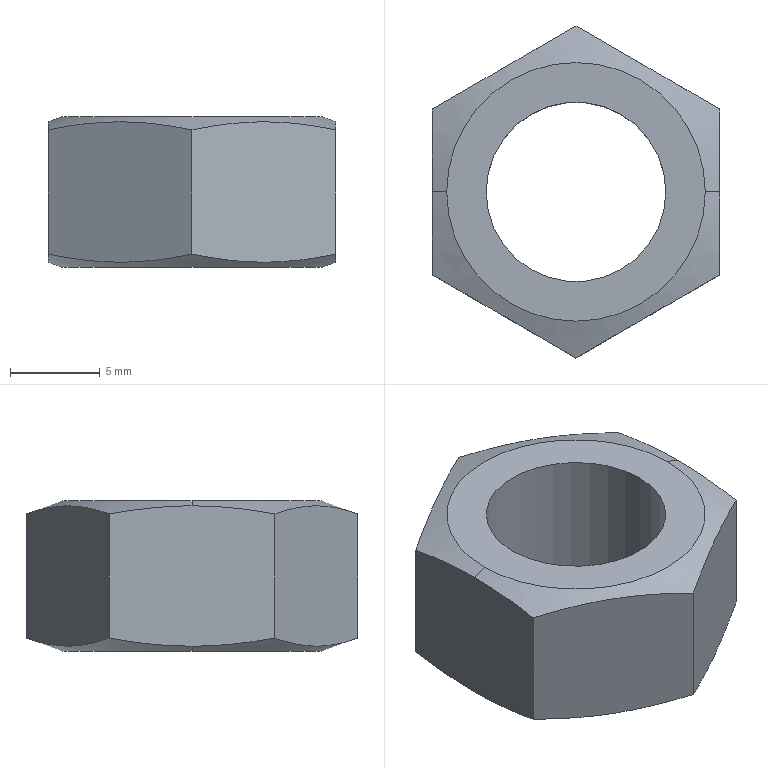Component | SolidWorks | HexNutM10-11 | 1 solid | 14 faces | box 16 x 18.48 x 8.4 mm | volume 1174 mm3 | plane 8 | cone 4 | cylinder 2 | commonest cylinder face diameters 10 x2
build123d program:
from build123d import *

# Parameters (mm, degrees)
BOSS_EXTRUDE1_DEPTH = 8.4
SKETCH5_R           = 5
CUT_EXTRUDE1_DEPTH  = 15.829


with BuildPart() as part:
    # Sketch1 → Boss-Extrude1 (new body)
    with BuildSketch(Plane.XY):
        Polygon((0, 9.238), (-8, 4.619), (-8, -4.619), (0, -9.238), (8, -4.619), (8, 4.619), align=None)
    extrude(amount=BOSS_EXTRUDE1_DEPTH)

    # Sketch4 → Cut-Revolve1 (revolve, cut)
    with BuildSketch(Plane(origin=(0, 0, 0), x_dir=(0, 0, -1), z_dir=(1, 0, 0)), mode=Mode.PRIVATE) as cut_revolve1_sk:
        Polygon((-8.4, -7.2), (-7.658, -9.238), (-8.4, -9.238), align=None)
    cut_revolve1 = revolve(cut_revolve1_sk.sketch.rotate(Axis((0, 0, 8.4), (0, 0, -1)), 120), axis=Axis((0, 0, 8.4), (0, 0, -1)), mode=Mode.SUBTRACT)

    # Mirror1: Cut-Revolve1 across plane
    add(cut_revolve1.mirror(Plane.XY.offset(4.2)), mode=Mode.SUBTRACT)

    # Sketch5 → Cut-Extrude1 (cut, through all)
    with BuildSketch(Plane.XY.offset(8.4)):
        Circle(SKETCH5_R)
    extrude(amount=-CUT_EXTRUDE1_DEPTH, mode=Mode.SUBTRACT)


solid = part.part

# Placed as in the assembly
solid = solid.moved(Location((-5489.995, 7146.665, 122.592), (0, 0, 0)))
STEP:
#1=COLOUR_RGB('',0.7922,0.8196,0.9333);
#2=FILL_AREA_STYLE_COLOUR('',#1);
#3=FILL_AREA_STYLE('',(#2));
#4=SURFACE_STYLE_FILL_AREA(#3);
#5=SURFACE_SIDE_STYLE('',(#4));
#6=SURFACE_STYLE_USAGE(.BOTH.,#5);
#7=PRESENTATION_STYLE_ASSIGNMENT((#6));
#8=CARTESIAN_POINT('',(-216.338,281.365,4.826));
#9=VERTEX_POINT('',#8);
#10=CARTESIAN_POINT('',(-215.945,281.365,4.826));
#11=VERTEX_POINT('',#10);
#12=CARTESIAN_POINT('',(-216.142,281.365,4.826));
#13=DIRECTION('',(0.,0.,1.));
#14=DIRECTION('',(1.,0.,0.));
#15=AXIS2_PLACEMENT_3D('',#12,#13,#14);
#16=CIRCLE('',#15,0.1969);
#17=EDGE_CURVE('',#9,#11,#16,.T.);
#18=ORIENTED_EDGE('',*,*,#17,.F.);
#19=CARTESIAN_POINT('',(-216.338,281.365,5.157));
#20=VERTEX_POINT('',#19);
#21=CARTESIAN_POINT('',(-216.338,281.365,4.826));
#22=DIRECTION('',(0.,0.,1.));
#23=VECTOR('',#22,39.37);
#24=LINE('',#21,#23);
#25=EDGE_CURVE('',#9,#20,#24,.T.);
#26=ORIENTED_EDGE('',*,*,#25,.T.);
#27=CARTESIAN_POINT('',(-215.945,281.365,5.157));
#28=VERTEX_POINT('',#27);
#29=CARTESIAN_POINT('',(-216.142,281.365,5.157));
#30=DIRECTION('',(0.,0.,1.));
#31=DIRECTION('',(1.,0.,0.));
#32=AXIS2_PLACEMENT_3D('',#29,#30,#31);
#33=CIRCLE('',#32,0.1969);
#34=EDGE_CURVE('',#20,#28,#33,.T.);
#35=ORIENTED_EDGE('',*,*,#34,.T.);
#36=CARTESIAN_POINT('',(-215.945,281.365,4.826));
#37=DIRECTION('',(0.,0.,1.));
#38=VECTOR('',#37,39.37);
#39=LINE('',#36,#38);
#40=EDGE_CURVE('',#11,#28,#39,.T.);
#41=ORIENTED_EDGE('',*,*,#40,.F.);
#42=EDGE_LOOP('',(#18,#26,#35,#41));
#43=FACE_OUTER_BOUND('',#42,.T.);
#44=CARTESIAN_POINT('',(-216.142,281.365,4.826));
#45=DIRECTION('',(0.,0.,1.));
#46=DIRECTION('',(1.,0.,0.));
#47=AXIS2_PLACEMENT_3D('',#44,#45,#46);
#48=CYLINDRICAL_SURFACE('',#47,0.1969);
#49=ADVANCED_FACE('',(#43),#48,.F.);
#50=CARTESIAN_POINT('',(-216.425,281.365,4.826));
#51=VERTEX_POINT('',#50);
#52=CARTESIAN_POINT('',(-215.858,281.365,4.826));
#53=VERTEX_POINT('',#52);
#54=CARTESIAN_POINT('',(-216.142,281.365,4.826));
#55=DIRECTION('',(0.,0.,1.));
#56=DIRECTION('',(1.,0.,0.));
#57=AXIS2_PLACEMENT_3D('',#54,#55,#56);
#58=CIRCLE('',#57,0.2835);
#59=EDGE_CURVE('',#51,#53,#58,.T.);
#60=ORIENTED_EDGE('',*,*,#59,.T.);
#61=CARTESIAN_POINT('',(-215.827,281.365,4.838));
#62=VERTEX_POINT('',#61);
#63=CARTESIAN_POINT('',(-215.778,281.365,4.856));
#64=DIRECTION('',(0.9397,-0.,0.342));
#65=VECTOR('',#64,39.37);
#66=LINE('',#63,#65);
#67=EDGE_CURVE('',#53,#62,#66,.T.);
#68=ORIENTED_EDGE('',*,*,#67,.T.);
#69=CARTESIAN_POINT('',(-215.827,281.183,4.856));
#70=VERTEX_POINT('',#69);
#71=CARTESIAN_POINT('',(-215.827,281.183,4.856));
#72=CARTESIAN_POINT('',(-215.827,281.213,4.85));
#73=CARTESIAN_POINT('',(-215.827,281.243,4.846));
#74=CARTESIAN_POINT('',(-215.827,281.304,4.84));
#75=CARTESIAN_POINT('',(-215.827,281.334,4.838));
#76=CARTESIAN_POINT('',(-215.827,281.365,4.838));
#77=B_SPLINE_CURVE_WITH_KNOTS('',3,(#71,#72,#73,#74,#75,#76),.UNSPECIFIED.,.F.,.F.,(4,2,4),(0.007828,0.01016,0.01248),.UNSPECIFIED.);
#78=EDGE_CURVE('',#70,#62,#77,.T.);
#79=ORIENTED_EDGE('',*,*,#78,.F.);
#80=CARTESIAN_POINT('',(-216.142,281.001,4.856));
#81=VERTEX_POINT('',#80);
#82=CARTESIAN_POINT('',(-216.142,281.001,4.856));
#83=CARTESIAN_POINT('',(-216.115,281.016,4.85));
#84=CARTESIAN_POINT('',(-216.089,281.031,4.846));
#85=CARTESIAN_POINT('',(-216.037,281.062,4.84));
#86=CARTESIAN_POINT('',(-215.984,281.092,4.836));
#87=CARTESIAN_POINT('',(-215.932,281.122,4.84));
#88=CARTESIAN_POINT('',(-215.879,281.153,4.846));
#89=CARTESIAN_POINT('',(-215.853,281.168,4.85));
#90=CARTESIAN_POINT('',(-215.827,281.183,4.856));
#91=B_SPLINE_CURVE_WITH_KNOTS('',3,(#82,#83,#84,#85,#86,#87,#88,#89,#90),.UNSPECIFIED.,.F.,.F.,(4,2,1,2,4),(0.00000023,0.00231,0.004619,0.006928,0.009238),.UNSPECIFIED.);
#92=EDGE_CURVE('',#81,#70,#91,.T.);
#93=ORIENTED_EDGE('',*,*,#92,.F.);
#94=CARTESIAN_POINT('',(-216.456,281.183,4.856));
#95=VERTEX_POINT('',#94);
#96=CARTESIAN_POINT('',(-216.456,281.183,4.856));
#97=CARTESIAN_POINT('',(-216.43,281.168,4.85));
#98=CARTESIAN_POINT('',(-216.404,281.153,4.846));
#99=CARTESIAN_POINT('',(-216.351,281.122,4.84));
#100=CARTESIAN_POINT('',(-216.299,281.092,4.836));
#101=CARTESIAN_POINT('',(-216.247,281.062,4.84));
#102=CARTESIAN_POINT('',(-216.194,281.031,4.846));
#103=CARTESIAN_POINT('',(-216.168,281.016,4.85));
#104=CARTESIAN_POINT('',(-216.142,281.001,4.856));
#105=B_SPLINE_CURVE_WITH_KNOTS('',3,(#96,#97,#98,#99,#100,#101,#102,#103,#104),.UNSPECIFIED.,.F.,.F.,(4,2,1,2,4),(0.00000023,0.00231,0.004619,0.006928,0.009238),.UNSPECIFIED.);
#106=EDGE_CURVE('',#95,#81,#105,.T.);
#107=ORIENTED_EDGE('',*,*,#106,.F.);
#108=CARTESIAN_POINT('',(-216.456,281.365,4.838));
#109=VERTEX_POINT('',#108);
#110=CARTESIAN_POINT('',(-216.456,281.365,4.838));
#111=CARTESIAN_POINT('',(-216.456,281.334,4.838));
#112=CARTESIAN_POINT('',(-216.456,281.304,4.84));
#113=CARTESIAN_POINT('',(-216.456,281.243,4.846));
#114=CARTESIAN_POINT('',(-216.456,281.213,4.85));
#115=CARTESIAN_POINT('',(-216.456,281.183,4.856));
#116=B_SPLINE_CURVE_WITH_KNOTS('',3,(#110,#111,#112,#113,#114,#115),.UNSPECIFIED.,.F.,.F.,(4,2,4),(0.02142,0.02374,0.02606),.UNSPECIFIED.);
#117=EDGE_CURVE('',#109,#95,#116,.T.);
#118=ORIENTED_EDGE('',*,*,#117,.F.);
#119=CARTESIAN_POINT('',(-216.505,281.365,4.856));
#120=DIRECTION('',(-0.9397,0.,0.342));
#121=VECTOR('',#120,39.37);
#122=LINE('',#119,#121);
#123=EDGE_CURVE('',#51,#109,#122,.T.);
#124=ORIENTED_EDGE('',*,*,#123,.F.);
#125=EDGE_LOOP('',(#60,#68,#79,#93,#107,#118,#124));
#126=FACE_OUTER_BOUND('',#125,.T.);
#127=CARTESIAN_POINT('',(-216.142,281.365,4.856));
#128=DIRECTION('',(0.,0.,1.));
#129=DIRECTION('',(-1.,0.,0.));
#130=AXIS2_PLACEMENT_3D('',#127,#128,#129);
#131=CONICAL_SURFACE('',#130,0.3637,1.222);
#132=ADVANCED_FACE('',(#126),#131,.T.);
#133=CARTESIAN_POINT('',(-215.858,281.365,5.157));
#134=VERTEX_POINT('',#133);
#135=CARTESIAN_POINT('',(-216.425,281.365,5.157));
#136=VERTEX_POINT('',#135);
#137=CARTESIAN_POINT('',(-216.142,281.365,5.157));
#138=DIRECTION('',(0.,0.,1.));
#139=DIRECTION('',(1.,0.,0.));
#140=AXIS2_PLACEMENT_3D('',#137,#138,#139);
#141=CIRCLE('',#140,0.2835);
#142=EDGE_CURVE('',#134,#136,#141,.T.);
#143=ORIENTED_EDGE('',*,*,#142,.F.);
#144=CARTESIAN_POINT('',(-215.827,281.365,5.146));
#145=VERTEX_POINT('',#144);
#146=CARTESIAN_POINT('',(-215.778,281.365,5.128));
#147=DIRECTION('',(0.9397,0.,-0.342));
#148=VECTOR('',#147,39.37);
#149=LINE('',#146,#148);
#150=EDGE_CURVE('',#134,#145,#149,.T.);
#151=ORIENTED_EDGE('',*,*,#150,.T.);
#152=CARTESIAN_POINT('',(-215.827,281.547,5.128));
#153=VERTEX_POINT('',#152);
#154=CARTESIAN_POINT('',(-215.827,281.547,5.128));
#155=CARTESIAN_POINT('',(-215.827,281.516,5.133));
#156=CARTESIAN_POINT('',(-215.827,281.486,5.138));
#157=CARTESIAN_POINT('',(-215.827,281.425,5.144));
#158=CARTESIAN_POINT('',(-215.827,281.395,5.146));
#159=CARTESIAN_POINT('',(-215.827,281.365,5.146));
#160=B_SPLINE_CURVE_WITH_KNOTS('',3,(#154,#155,#156,#157,#158,#159),.UNSPECIFIED.,.F.,.F.,(4,2,4),(0.01676,0.01909,0.02142),.UNSPECIFIED.);
#161=EDGE_CURVE('',#153,#145,#160,.T.);
#162=ORIENTED_EDGE('',*,*,#161,.F.);
#163=CARTESIAN_POINT('',(-216.142,281.728,5.128));
#164=VERTEX_POINT('',#163);
#165=CARTESIAN_POINT('',(-216.142,281.728,5.128));
#166=CARTESIAN_POINT('',(-216.115,281.713,5.133));
#167=CARTESIAN_POINT('',(-216.089,281.698,5.138));
#168=CARTESIAN_POINT('',(-216.037,281.668,5.144));
#169=CARTESIAN_POINT('',(-215.984,281.638,5.147));
#170=CARTESIAN_POINT('',(-215.932,281.607,5.144));
#171=CARTESIAN_POINT('',(-215.879,281.577,5.138));
#172=CARTESIAN_POINT('',(-215.853,281.562,5.133));
#173=CARTESIAN_POINT('',(-215.827,281.547,5.128));
#174=B_SPLINE_CURVE_WITH_KNOTS('',3,(#165,#166,#167,#168,#169,#170,#171,#172,#173),.UNSPECIFIED.,.F.,.F.,(4,2,1,2,4),(0.00000023,0.00231,0.004619,0.006928,0.009238),.UNSPECIFIED.);
#175=EDGE_CURVE('',#164,#153,#174,.T.);
#176=ORIENTED_EDGE('',*,*,#175,.F.);
#177=CARTESIAN_POINT('',(-216.456,281.547,5.128));
#178=VERTEX_POINT('',#177);
#179=CARTESIAN_POINT('',(-216.456,281.547,5.128));
#180=CARTESIAN_POINT('',(-216.43,281.562,5.133));
#181=CARTESIAN_POINT('',(-216.404,281.577,5.138));
#182=CARTESIAN_POINT('',(-216.351,281.607,5.144));
#183=CARTESIAN_POINT('',(-216.299,281.638,5.147));
#184=CARTESIAN_POINT('',(-216.247,281.668,5.144));
#185=CARTESIAN_POINT('',(-216.194,281.698,5.138));
#186=CARTESIAN_POINT('',(-216.168,281.713,5.133));
#187=CARTESIAN_POINT('',(-216.142,281.728,5.128));
#188=B_SPLINE_CURVE_WITH_KNOTS('',3,(#179,#180,#181,#182,#183,#184,#185,#186,#187),.UNSPECIFIED.,.F.,.F.,(4,2,1,2,4),(0.00000023,0.00231,0.004619,0.006928,0.009238),.UNSPECIFIED.);
#189=EDGE_CURVE('',#178,#164,#188,.T.);
#190=ORIENTED_EDGE('',*,*,#189,.F.);
#191=CARTESIAN_POINT('',(-216.456,281.365,5.146));
#192=VERTEX_POINT('',#191);
#193=CARTESIAN_POINT('',(-216.456,281.365,5.146));
#194=CARTESIAN_POINT('',(-216.456,281.395,5.146));
#195=CARTESIAN_POINT('',(-216.456,281.425,5.144));
#196=CARTESIAN_POINT('',(-216.456,281.486,5.138));
#197=CARTESIAN_POINT('',(-216.456,281.516,5.133));
#198=CARTESIAN_POINT('',(-216.456,281.547,5.128));
#199=B_SPLINE_CURVE_WITH_KNOTS('',3,(#193,#194,#195,#196,#197,#198),.UNSPECIFIED.,.F.,.F.,(4,2,4),(0.01248,0.01482,0.01715),.UNSPECIFIED.);
#200=EDGE_CURVE('',#192,#178,#199,.T.);
#201=ORIENTED_EDGE('',*,*,#200,.F.);
#202=CARTESIAN_POINT('',(-216.505,281.365,5.128));
#203=DIRECTION('',(-0.9397,0.,-0.342));
#204=VECTOR('',#203,39.37);
#205=LINE('',#202,#204);
#206=EDGE_CURVE('',#136,#192,#205,.T.);
#207=ORIENTED_EDGE('',*,*,#206,.F.);
#208=EDGE_LOOP('',(#143,#151,#162,#176,#190,#201,#207));
#209=FACE_OUTER_BOUND('',#208,.T.);
#210=CARTESIAN_POINT('',(-216.142,281.365,5.128));
#211=DIRECTION('',(0.,0.,-1.));
#212=DIRECTION('',(-1.,0.,0.));
#213=AXIS2_PLACEMENT_3D('',#210,#211,#212);
#214=CONICAL_SURFACE('',#213,0.3637,1.222);
#215=ADVANCED_FACE('',(#209),#214,.T.);
#216=CARTESIAN_POINT('',(-215.827,281.547,4.856));
#217=VERTEX_POINT('',#216);
#218=CARTESIAN_POINT('',(-215.827,281.547,5.157));
#219=DIRECTION('',(0.,0.,-1.));
#220=VECTOR('',#219,39.37);
#221=LINE('',#218,#220);
#222=EDGE_CURVE('',#153,#217,#221,.T.);
#223=ORIENTED_EDGE('',*,*,#222,.T.);
#224=CARTESIAN_POINT('',(-216.142,281.728,4.856));
#225=VERTEX_POINT('',#224);
#226=CARTESIAN_POINT('',(-215.827,281.547,4.856));
#227=CARTESIAN_POINT('',(-215.853,281.562,4.85));
#228=CARTESIAN_POINT('',(-215.879,281.577,4.846));
#229=CARTESIAN_POINT('',(-215.932,281.607,4.84));
#230=CARTESIAN_POINT('',(-215.984,281.638,4.836));
#231=CARTESIAN_POINT('',(-216.037,281.668,4.84));
#232=CARTESIAN_POINT('',(-216.089,281.698,4.846));
#233=CARTESIAN_POINT('',(-216.115,281.713,4.85));
#234=CARTESIAN_POINT('',(-216.142,281.728,4.856));
#235=B_SPLINE_CURVE_WITH_KNOTS('',3,(#226,#227,#228,#229,#230,#231,#232,#233,#234),.UNSPECIFIED.,.F.,.F.,(4,2,1,2,4),(0.00000023,0.00231,0.004619,0.006928,0.009238),.UNSPECIFIED.);
#236=EDGE_CURVE('',#217,#225,#235,.T.);
#237=ORIENTED_EDGE('',*,*,#236,.T.);
#238=CARTESIAN_POINT('',(-216.142,281.728,5.157));
#239=DIRECTION('',(0.,0.,-1.));
#240=VECTOR('',#239,39.37);
#241=LINE('',#238,#240);
#242=EDGE_CURVE('',#164,#225,#241,.T.);
#243=ORIENTED_EDGE('',*,*,#242,.F.);
#244=ORIENTED_EDGE('',*,*,#175,.T.);
#245=EDGE_LOOP('',(#223,#237,#243,#244));
#246=FACE_OUTER_BOUND('',#245,.T.);
#247=CARTESIAN_POINT('',(-215.827,281.547,5.157));
#248=DIRECTION('',(-0.5,-0.866,0.));
#249=DIRECTION('',(0.866,-0.5,0.));
#250=AXIS2_PLACEMENT_3D('',#247,#248,#249);
#251=PLANE('',#250);
#252=ADVANCED_FACE('',(#246),#251,.F.);
#253=ORIENTED_EDGE('',*,*,#242,.T.);
#254=CARTESIAN_POINT('',(-216.456,281.547,4.856));
#255=VERTEX_POINT('',#254);
#256=CARTESIAN_POINT('',(-216.142,281.728,4.856));
#257=CARTESIAN_POINT('',(-216.168,281.713,4.85));
#258=CARTESIAN_POINT('',(-216.194,281.698,4.846));
#259=CARTESIAN_POINT('',(-216.247,281.668,4.84));
#260=CARTESIAN_POINT('',(-216.299,281.638,4.836));
#261=CARTESIAN_POINT('',(-216.351,281.607,4.84));
#262=CARTESIAN_POINT('',(-216.404,281.577,4.846));
#263=CARTESIAN_POINT('',(-216.43,281.562,4.85));
#264=CARTESIAN_POINT('',(-216.456,281.547,4.856));
#265=B_SPLINE_CURVE_WITH_KNOTS('',3,(#256,#257,#258,#259,#260,#261,#262,#263,#264),.UNSPECIFIED.,.F.,.F.,(4,2,1,2,4),(0.00000023,0.00231,0.004619,0.006928,0.009238),.UNSPECIFIED.);
#266=EDGE_CURVE('',#225,#255,#265,.T.);
#267=ORIENTED_EDGE('',*,*,#266,.T.);
#268=CARTESIAN_POINT('',(-216.456,281.547,5.157));
#269=DIRECTION('',(0.,0.,-1.));
#270=VECTOR('',#269,39.37);
#271=LINE('',#268,#270);
#272=EDGE_CURVE('',#178,#255,#271,.T.);
#273=ORIENTED_EDGE('',*,*,#272,.F.);
#274=ORIENTED_EDGE('',*,*,#189,.T.);
#275=EDGE_LOOP('',(#253,#267,#273,#274));
#276=FACE_OUTER_BOUND('',#275,.T.);
#277=CARTESIAN_POINT('',(-216.142,281.728,5.157));
#278=DIRECTION('',(0.5,-0.866,0.));
#279=DIRECTION('',(0.866,0.5,0.));
#280=AXIS2_PLACEMENT_3D('',#277,#278,#279);
#281=PLANE('',#280);
#282=ADVANCED_FACE('',(#276),#281,.F.);
#283=ORIENTED_EDGE('',*,*,#272,.T.);
#284=CARTESIAN_POINT('',(-216.456,281.547,4.856));
#285=CARTESIAN_POINT('',(-216.456,281.516,4.85));
#286=CARTESIAN_POINT('',(-216.456,281.486,4.846));
#287=CARTESIAN_POINT('',(-216.456,281.425,4.84));
#288=CARTESIAN_POINT('',(-216.456,281.395,4.838));
#289=CARTESIAN_POINT('',(-216.456,281.365,4.838));
#290=B_SPLINE_CURVE_WITH_KNOTS('',3,(#284,#285,#286,#287,#288,#289),.UNSPECIFIED.,.F.,.F.,(4,2,4),(0.01676,0.01909,0.02142),.UNSPECIFIED.);
#291=EDGE_CURVE('',#255,#109,#290,.T.);
#292=ORIENTED_EDGE('',*,*,#291,.T.);
#293=ORIENTED_EDGE('',*,*,#117,.T.);
#294=CARTESIAN_POINT('',(-216.456,281.183,5.128));
#295=VERTEX_POINT('',#294);
#296=CARTESIAN_POINT('',(-216.456,281.183,5.157));
#297=DIRECTION('',(0.,0.,-1.));
#298=VECTOR('',#297,39.37);
#299=LINE('',#296,#298);
#300=EDGE_CURVE('',#295,#95,#299,.T.);
#301=ORIENTED_EDGE('',*,*,#300,.F.);
#302=CARTESIAN_POINT('',(-216.456,281.183,5.128));
#303=CARTESIAN_POINT('',(-216.456,281.213,5.133));
#304=CARTESIAN_POINT('',(-216.456,281.243,5.138));
#305=CARTESIAN_POINT('',(-216.456,281.304,5.144));
#306=CARTESIAN_POINT('',(-216.456,281.334,5.146));
#307=CARTESIAN_POINT('',(-216.456,281.365,5.146));
#308=B_SPLINE_CURVE_WITH_KNOTS('',3,(#302,#303,#304,#305,#306,#307),.UNSPECIFIED.,.F.,.F.,(4,2,4),(0.007828,0.01016,0.01248),.UNSPECIFIED.);
#309=EDGE_CURVE('',#295,#192,#308,.T.);
#310=ORIENTED_EDGE('',*,*,#309,.T.);
#311=ORIENTED_EDGE('',*,*,#200,.T.);
#312=EDGE_LOOP('',(#283,#292,#293,#301,#310,#311));
#313=FACE_OUTER_BOUND('',#312,.T.);
#314=CARTESIAN_POINT('',(-216.456,281.547,5.157));
#315=DIRECTION('',(1.,0.,0.));
#316=DIRECTION('',(0.,0.,-1.));
#317=AXIS2_PLACEMENT_3D('',#314,#315,#316);
#318=PLANE('',#317);
#319=ADVANCED_FACE('',(#313),#318,.F.);
#320=ORIENTED_EDGE('',*,*,#300,.T.);
#321=ORIENTED_EDGE('',*,*,#106,.T.);
#322=CARTESIAN_POINT('',(-216.142,281.001,5.128));
#323=VERTEX_POINT('',#322);
#324=CARTESIAN_POINT('',(-216.142,281.001,5.157));
#325=DIRECTION('',(0.,0.,-1.));
#326=VECTOR('',#325,39.37);
#327=LINE('',#324,#326);
#328=EDGE_CURVE('',#323,#81,#327,.T.);
#329=ORIENTED_EDGE('',*,*,#328,.F.);
#330=CARTESIAN_POINT('',(-216.142,281.001,5.128));
#331=CARTESIAN_POINT('',(-216.168,281.016,5.133));
#332=CARTESIAN_POINT('',(-216.194,281.031,5.138));
#333=CARTESIAN_POINT('',(-216.247,281.062,5.144));
#334=CARTESIAN_POINT('',(-216.299,281.092,5.147));
#335=CARTESIAN_POINT('',(-216.351,281.122,5.144));
#336=CARTESIAN_POINT('',(-216.404,281.153,5.138));
#337=CARTESIAN_POINT('',(-216.43,281.168,5.133));
#338=CARTESIAN_POINT('',(-216.456,281.183,5.128));
#339=B_SPLINE_CURVE_WITH_KNOTS('',3,(#330,#331,#332,#333,#334,#335,#336,#337,#338),.UNSPECIFIED.,.F.,.F.,(4,2,1,2,4),(0.00000023,0.00231,0.004619,0.006928,0.009238),.UNSPECIFIED.);
#340=EDGE_CURVE('',#323,#295,#339,.T.);
#341=ORIENTED_EDGE('',*,*,#340,.T.);
#342=EDGE_LOOP('',(#320,#321,#329,#341));
#343=FACE_OUTER_BOUND('',#342,.T.);
#344=CARTESIAN_POINT('',(-216.456,281.183,5.157));
#345=DIRECTION('',(0.5,0.866,0.));
#346=DIRECTION('',(-0.866,0.5,0.));
#347=AXIS2_PLACEMENT_3D('',#344,#345,#346);
#348=PLANE('',#347);
#349=ADVANCED_FACE('',(#343),#348,.F.);
#350=ORIENTED_EDGE('',*,*,#328,.T.);
#351=ORIENTED_EDGE('',*,*,#92,.T.);
#352=CARTESIAN_POINT('',(-215.827,281.183,5.128));
#353=VERTEX_POINT('',#352);
#354=CARTESIAN_POINT('',(-215.827,281.183,5.157));
#355=DIRECTION('',(0.,0.,-1.));
#356=VECTOR('',#355,39.37);
#357=LINE('',#354,#356);
#358=EDGE_CURVE('',#353,#70,#357,.T.);
#359=ORIENTED_EDGE('',*,*,#358,.F.);
#360=CARTESIAN_POINT('',(-215.827,281.183,5.128));
#361=CARTESIAN_POINT('',(-215.853,281.168,5.133));
#362=CARTESIAN_POINT('',(-215.879,281.153,5.138));
#363=CARTESIAN_POINT('',(-215.932,281.122,5.144));
#364=CARTESIAN_POINT('',(-215.984,281.092,5.147));
#365=CARTESIAN_POINT('',(-216.037,281.062,5.144));
#366=CARTESIAN_POINT('',(-216.089,281.031,5.138));
#367=CARTESIAN_POINT('',(-216.115,281.016,5.133));
#368=CARTESIAN_POINT('',(-216.142,281.001,5.128));
#369=B_SPLINE_CURVE_WITH_KNOTS('',3,(#360,#361,#362,#363,#364,#365,#366,#367,#368),.UNSPECIFIED.,.F.,.F.,(4,2,1,2,4),(0.00000023,0.00231,0.004619,0.006928,0.009238),.UNSPECIFIED.);
#370=EDGE_CURVE('',#353,#323,#369,.T.);
#371=ORIENTED_EDGE('',*,*,#370,.T.);
#372=EDGE_LOOP('',(#350,#351,#359,#371));
#373=FACE_OUTER_BOUND('',#372,.T.);
#374=CARTESIAN_POINT('',(-216.142,281.001,5.157));
#375=DIRECTION('',(-0.5,0.866,0.));
#376=DIRECTION('',(-0.866,-0.5,0.));
#377=AXIS2_PLACEMENT_3D('',#374,#375,#376);
#378=PLANE('',#377);
#379=ADVANCED_FACE('',(#373),#378,.F.);
#380=ORIENTED_EDGE('',*,*,#358,.T.);
#381=ORIENTED_EDGE('',*,*,#78,.T.);
#382=CARTESIAN_POINT('',(-215.827,281.365,4.838));
#383=CARTESIAN_POINT('',(-215.827,281.395,4.838));
#384=CARTESIAN_POINT('',(-215.827,281.425,4.84));
#385=CARTESIAN_POINT('',(-215.827,281.486,4.846));
#386=CARTESIAN_POINT('',(-215.827,281.516,4.85));
#387=CARTESIAN_POINT('',(-215.827,281.547,4.856));
#388=B_SPLINE_CURVE_WITH_KNOTS('',3,(#382,#383,#384,#385,#386,#387),.UNSPECIFIED.,.F.,.F.,(4,2,4),(0.01248,0.01482,0.01715),.UNSPECIFIED.);
#389=EDGE_CURVE('',#62,#217,#388,.T.);
#390=ORIENTED_EDGE('',*,*,#389,.T.);
#391=ORIENTED_EDGE('',*,*,#222,.F.);
#392=ORIENTED_EDGE('',*,*,#161,.T.);
#393=CARTESIAN_POINT('',(-215.827,281.365,5.146));
#394=CARTESIAN_POINT('',(-215.827,281.334,5.146));
#395=CARTESIAN_POINT('',(-215.827,281.304,5.144));
#396=CARTESIAN_POINT('',(-215.827,281.243,5.138));
#397=CARTESIAN_POINT('',(-215.827,281.213,5.133));
#398=CARTESIAN_POINT('',(-215.827,281.183,5.128));
#399=B_SPLINE_CURVE_WITH_KNOTS('',3,(#393,#394,#395,#396,#397,#398),.UNSPECIFIED.,.F.,.F.,(4,2,4),(0.02142,0.02374,0.02606),.UNSPECIFIED.);
#400=EDGE_CURVE('',#145,#353,#399,.T.);
#401=ORIENTED_EDGE('',*,*,#400,.T.);
#402=EDGE_LOOP('',(#380,#381,#390,#391,#392,#401));
#403=FACE_OUTER_BOUND('',#402,.T.);
#404=CARTESIAN_POINT('',(-215.827,281.183,5.157));
#405=DIRECTION('',(-1.,-0.,0.));
#406=DIRECTION('',(0.,-1.,0.));
#407=AXIS2_PLACEMENT_3D('',#404,#405,#406);
#408=PLANE('',#407);
#409=ADVANCED_FACE('',(#403),#408,.F.);
#410=ORIENTED_EDGE('',*,*,#150,.F.);
#411=CARTESIAN_POINT('',(-216.142,281.365,5.157));
#412=DIRECTION('',(0.,0.,1.));
#413=DIRECTION('',(1.,0.,0.));
#414=AXIS2_PLACEMENT_3D('',#411,#412,#413);
#415=CIRCLE('',#414,0.2835);
#416=EDGE_CURVE('',#136,#134,#415,.T.);
#417=ORIENTED_EDGE('',*,*,#416,.F.);
#418=ORIENTED_EDGE('',*,*,#206,.T.);
#419=ORIENTED_EDGE('',*,*,#309,.F.);
#420=ORIENTED_EDGE('',*,*,#340,.F.);
#421=ORIENTED_EDGE('',*,*,#370,.F.);
#422=ORIENTED_EDGE('',*,*,#400,.F.);
#423=EDGE_LOOP('',(#410,#417,#418,#419,#420,#421,#422));
#424=FACE_OUTER_BOUND('',#423,.T.);
#425=CARTESIAN_POINT('',(-216.142,281.365,5.128));
#426=DIRECTION('',(0.,0.,-1.));
#427=DIRECTION('',(-1.,0.,0.));
#428=AXIS2_PLACEMENT_3D('',#425,#426,#427);
#429=CONICAL_SURFACE('',#428,0.3637,1.222);
#430=ADVANCED_FACE('',(#424),#429,.T.);
#431=CARTESIAN_POINT('',(-216.142,281.365,5.157));
#432=DIRECTION('',(0.,0.,1.));
#433=DIRECTION('',(1.,0.,0.));
#434=AXIS2_PLACEMENT_3D('',#431,#432,#433);
#435=CIRCLE('',#434,0.1969);
#436=EDGE_CURVE('',#28,#20,#435,.T.);
#437=ORIENTED_EDGE('',*,*,#436,.F.);
#438=ORIENTED_EDGE('',*,*,#34,.F.);
#439=EDGE_LOOP('',(#437,#438));
#440=FACE_BOUND('',#439,.T.);
#441=ORIENTED_EDGE('',*,*,#416,.T.);
#442=ORIENTED_EDGE('',*,*,#142,.T.);
#443=EDGE_LOOP('',(#441,#442));
#444=FACE_OUTER_BOUND('',#443,.T.);
#445=CARTESIAN_POINT('',(-216.142,281.365,5.157));
#446=DIRECTION('',(0.,0.,1.));
#447=DIRECTION('',(1.,0.,0.));
#448=AXIS2_PLACEMENT_3D('',#445,#446,#447);
#449=PLANE('',#448);
#450=ADVANCED_FACE('',(#440,#444),#449,.T.);
#451=ORIENTED_EDGE('',*,*,#67,.F.);
#452=CARTESIAN_POINT('',(-216.142,281.365,4.826));
#453=DIRECTION('',(0.,0.,1.));
#454=DIRECTION('',(1.,0.,0.));
#455=AXIS2_PLACEMENT_3D('',#452,#453,#454);
#456=CIRCLE('',#455,0.2835);
#457=EDGE_CURVE('',#53,#51,#456,.T.);
#458=ORIENTED_EDGE('',*,*,#457,.T.);
#459=ORIENTED_EDGE('',*,*,#123,.T.);
#460=ORIENTED_EDGE('',*,*,#291,.F.);
#461=ORIENTED_EDGE('',*,*,#266,.F.);
#462=ORIENTED_EDGE('',*,*,#236,.F.);
#463=ORIENTED_EDGE('',*,*,#389,.F.);
#464=EDGE_LOOP('',(#451,#458,#459,#460,#461,#462,#463));
#465=FACE_OUTER_BOUND('',#464,.T.);
#466=CARTESIAN_POINT('',(-216.142,281.365,4.856));
#467=DIRECTION('',(0.,0.,1.));
#468=DIRECTION('',(-1.,0.,0.));
#469=AXIS2_PLACEMENT_3D('',#466,#467,#468);
#470=CONICAL_SURFACE('',#469,0.3637,1.222);
#471=ADVANCED_FACE('',(#465),#470,.T.);
#472=CARTESIAN_POINT('',(-216.142,281.365,4.826));
#473=DIRECTION('',(0.,0.,1.));
#474=DIRECTION('',(1.,0.,0.));
#475=AXIS2_PLACEMENT_3D('',#472,#473,#474);
#476=CIRCLE('',#475,0.1969);
#477=EDGE_CURVE('',#11,#9,#476,.T.);
#478=ORIENTED_EDGE('',*,*,#477,.T.);
#479=ORIENTED_EDGE('',*,*,#17,.T.);
#480=EDGE_LOOP('',(#478,#479));
#481=FACE_BOUND('',#480,.T.);
#482=ORIENTED_EDGE('',*,*,#59,.F.);
#483=ORIENTED_EDGE('',*,*,#457,.F.);
#484=EDGE_LOOP('',(#482,#483));
#485=FACE_OUTER_BOUND('',#484,.T.);
#486=CARTESIAN_POINT('',(-216.142,281.365,4.826));
#487=DIRECTION('',(0.,0.,1.));
#488=DIRECTION('',(1.,0.,0.));
#489=AXIS2_PLACEMENT_3D('',#486,#487,#488);
#490=PLANE('',#489);
#491=ADVANCED_FACE('',(#481,#485),#490,.F.);
#492=ORIENTED_EDGE('',*,*,#25,.F.);
#493=ORIENTED_EDGE('',*,*,#477,.F.);
#494=ORIENTED_EDGE('',*,*,#40,.T.);
#495=ORIENTED_EDGE('',*,*,#436,.T.);
#496=EDGE_LOOP('',(#492,#493,#494,#495));
#497=FACE_OUTER_BOUND('',#496,.T.);
#498=CARTESIAN_POINT('',(-216.142,281.365,4.826));
#499=DIRECTION('',(0.,0.,1.));
#500=DIRECTION('',(1.,0.,0.));
#501=AXIS2_PLACEMENT_3D('',#498,#499,#500);
#502=CYLINDRICAL_SURFACE('',#501,0.1969);
#503=ADVANCED_FACE('',(#497),#502,.F.);
#504=CLOSED_SHELL('',(#49,#132,#215,#252,#282,#319,#349,#379,#409,#430,#450,#471,#491,#503));
#505=MANIFOLD_SOLID_BREP('',#504);
#506=STYLED_ITEM('',(#7),#505);
#507=PRESENTATION_LAYER_ASSIGNMENT('','',(#506));
#508=(LENGTH_UNIT()NAMED_UNIT(*)SI_UNIT($,.METRE.));
#509=LENGTH_MEASURE_WITH_UNIT(LENGTH_MEASURE(0.0254),#508);
#510=DIMENSIONAL_EXPONENTS(1.,0.,0.,0.,0.,0.,0.);
#511=(CONVERSION_BASED_UNIT('',#509)LENGTH_UNIT()NAMED_UNIT(#510));
#512=UNCERTAINTY_MEASURE_WITH_UNIT(LENGTH_MEASURE(0.00001),#511,'','');
#513=(NAMED_UNIT(*)PLANE_ANGLE_UNIT()SI_UNIT($,.RADIAN.));
#514=(NAMED_UNIT(*)SI_UNIT($,.STERADIAN.)SOLID_ANGLE_UNIT());
#515=(GEOMETRIC_REPRESENTATION_CONTEXT(3)GLOBAL_UNCERTAINTY_ASSIGNED_CONTEXT((#512))GLOBAL_UNIT_ASSIGNED_CONTEXT((#511,#513,#514))REPRESENTATION_CONTEXT('',''));
#516=MECHANICAL_DESIGN_GEOMETRIC_PRESENTATION_REPRESENTATION('',(#506),#515);
#517=CARTESIAN_POINT('',(0.,0.,0.));
#518=DIRECTION('',(0.,0.,1.));
#519=DIRECTION('',(1.,0.,0.));
#520=AXIS2_PLACEMENT_3D('',#517,#518,#519);
#521=(LENGTH_UNIT()NAMED_UNIT(*)SI_UNIT($,.METRE.));
#522=LENGTH_MEASURE_WITH_UNIT(LENGTH_MEASURE(0.0254),#521);
#523=DIMENSIONAL_EXPONENTS(1.,0.,0.,0.,0.,0.,0.);
#524=(CONVERSION_BASED_UNIT('',#522)LENGTH_UNIT()NAMED_UNIT(#523));
#525=UNCERTAINTY_MEASURE_WITH_UNIT(LENGTH_MEASURE(0.00001),#524,'','');
#526=(NAMED_UNIT(*)PLANE_ANGLE_UNIT()SI_UNIT($,.RADIAN.));
#527=(NAMED_UNIT(*)SI_UNIT($,.STERADIAN.)SOLID_ANGLE_UNIT());
#528=(GEOMETRIC_REPRESENTATION_CONTEXT(3)GLOBAL_UNCERTAINTY_ASSIGNED_CONTEXT((#525))GLOBAL_UNIT_ASSIGNED_CONTEXT((#524,#526,#527))REPRESENTATION_CONTEXT('',''));
#529=ADVANCED_BREP_SHAPE_REPRESENTATION('',(#505,#520),#528);